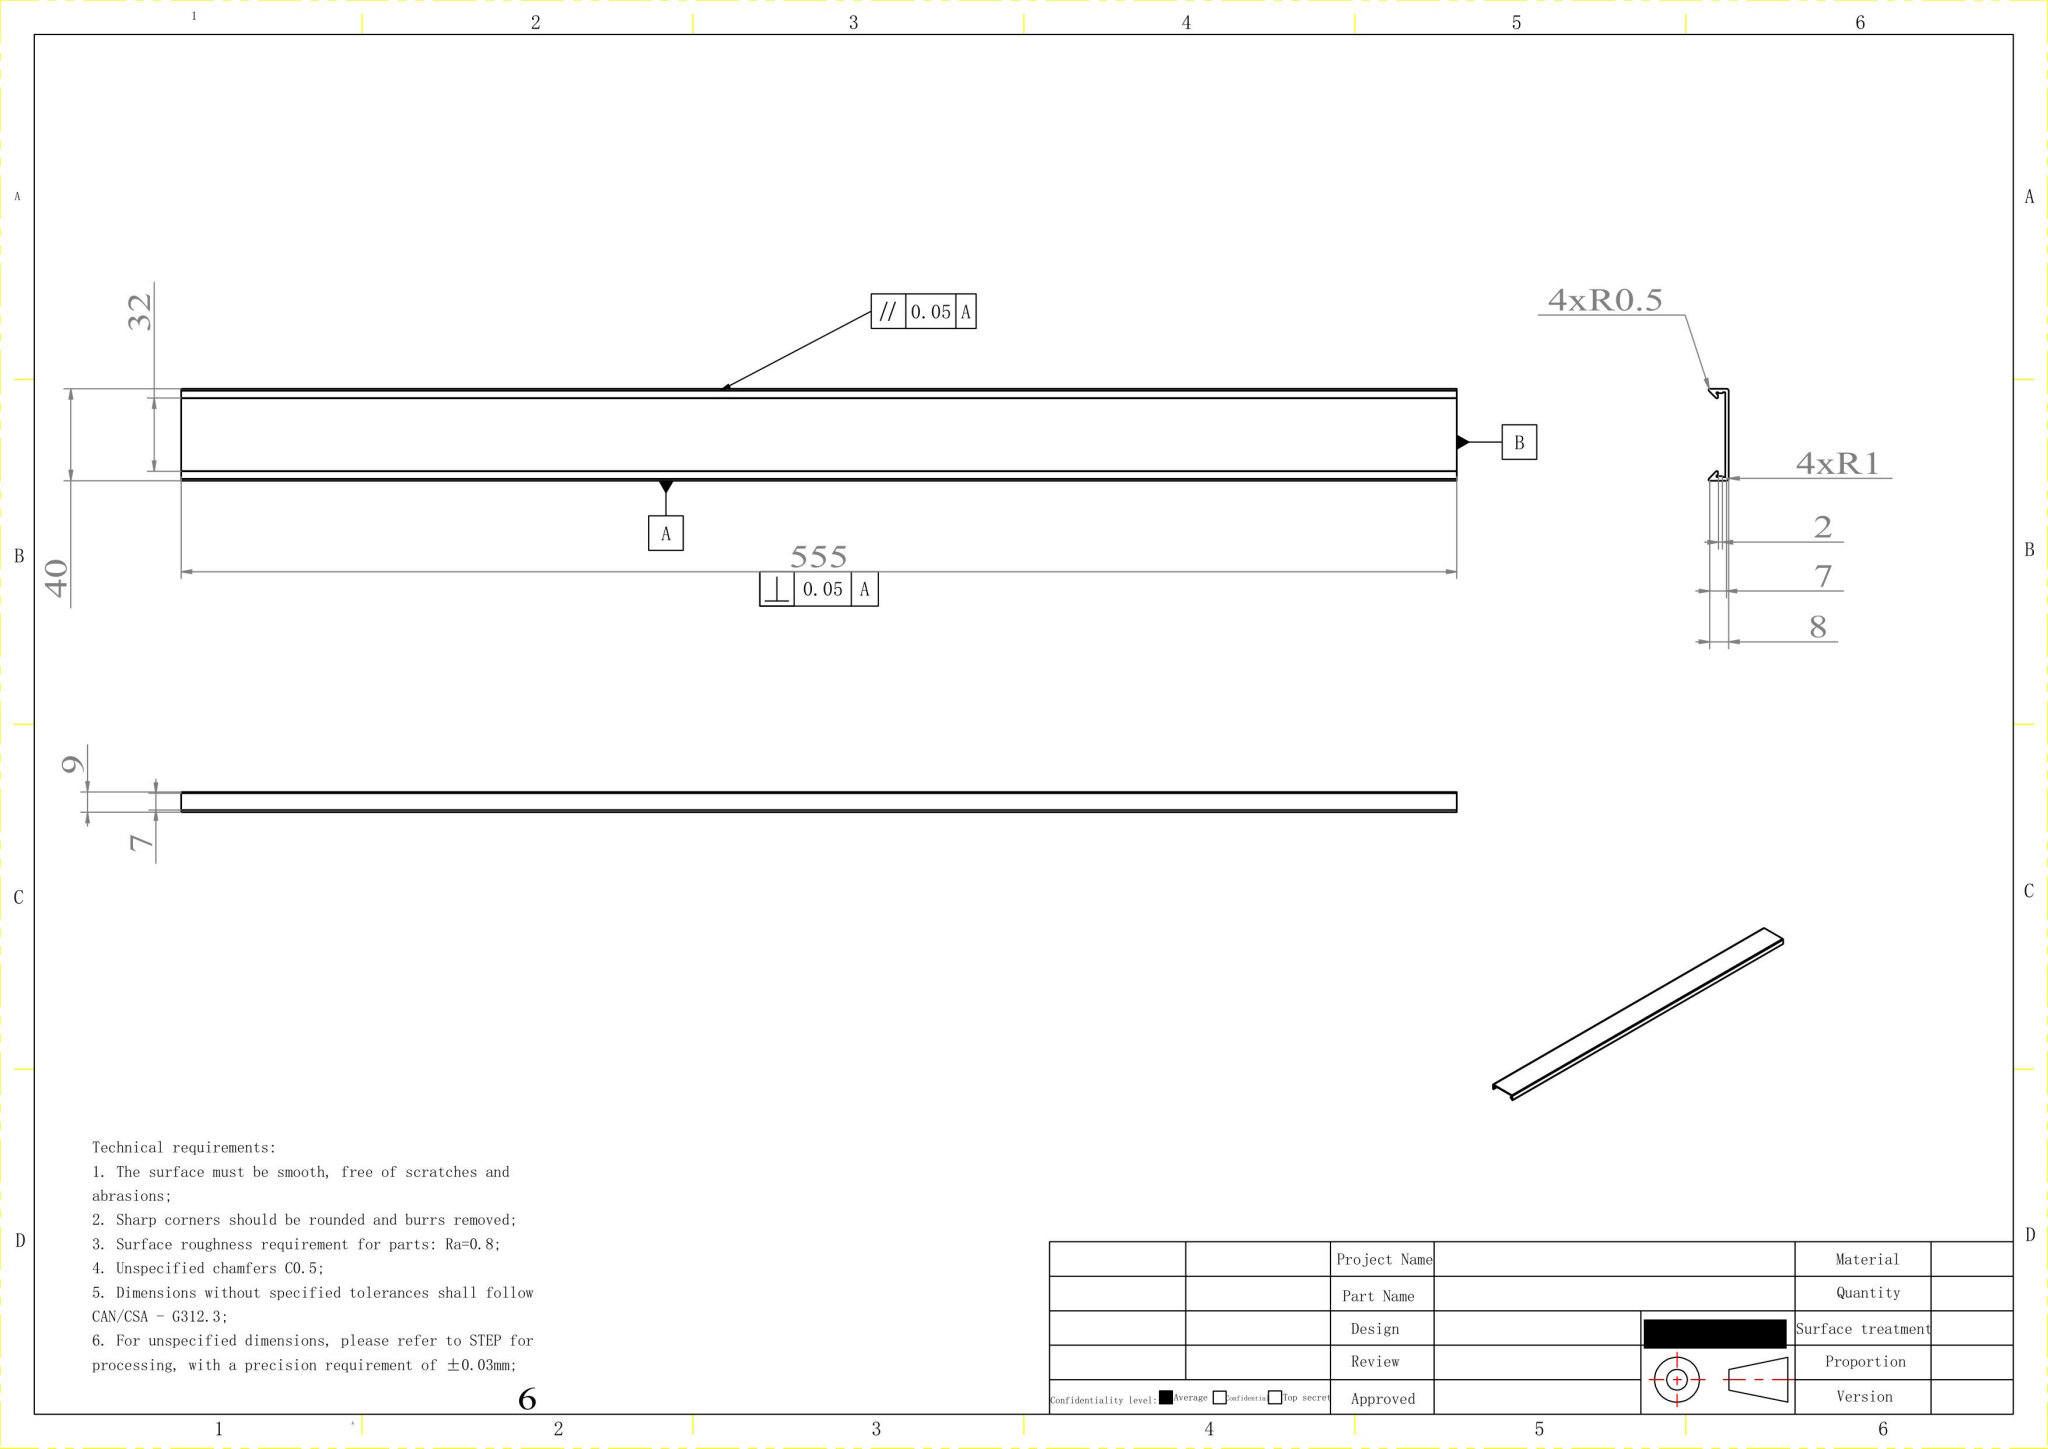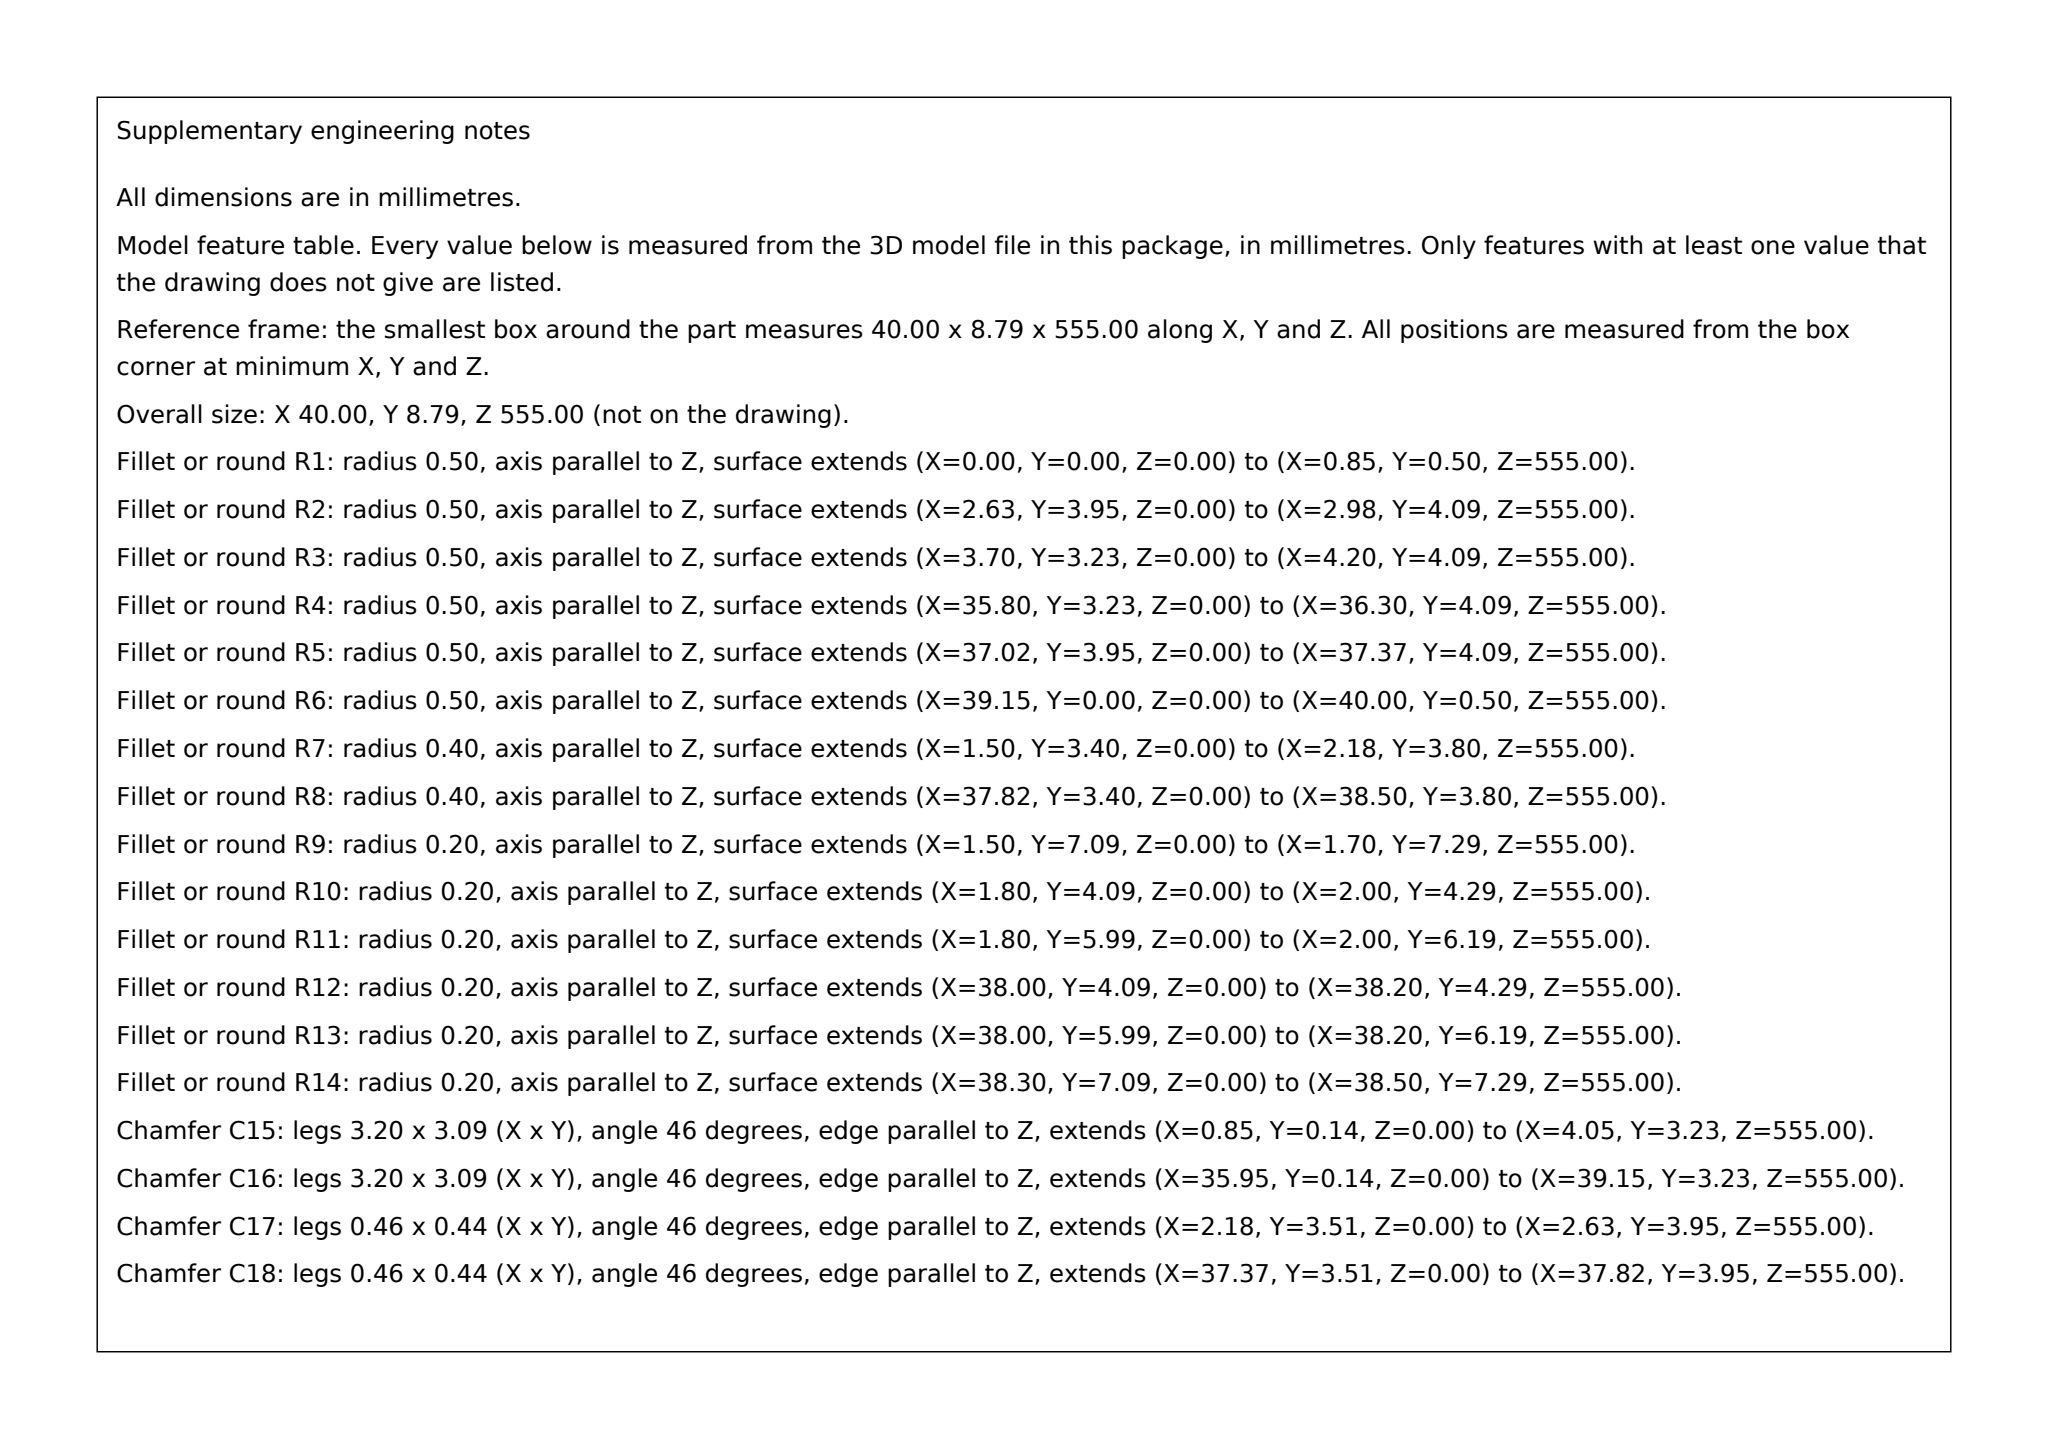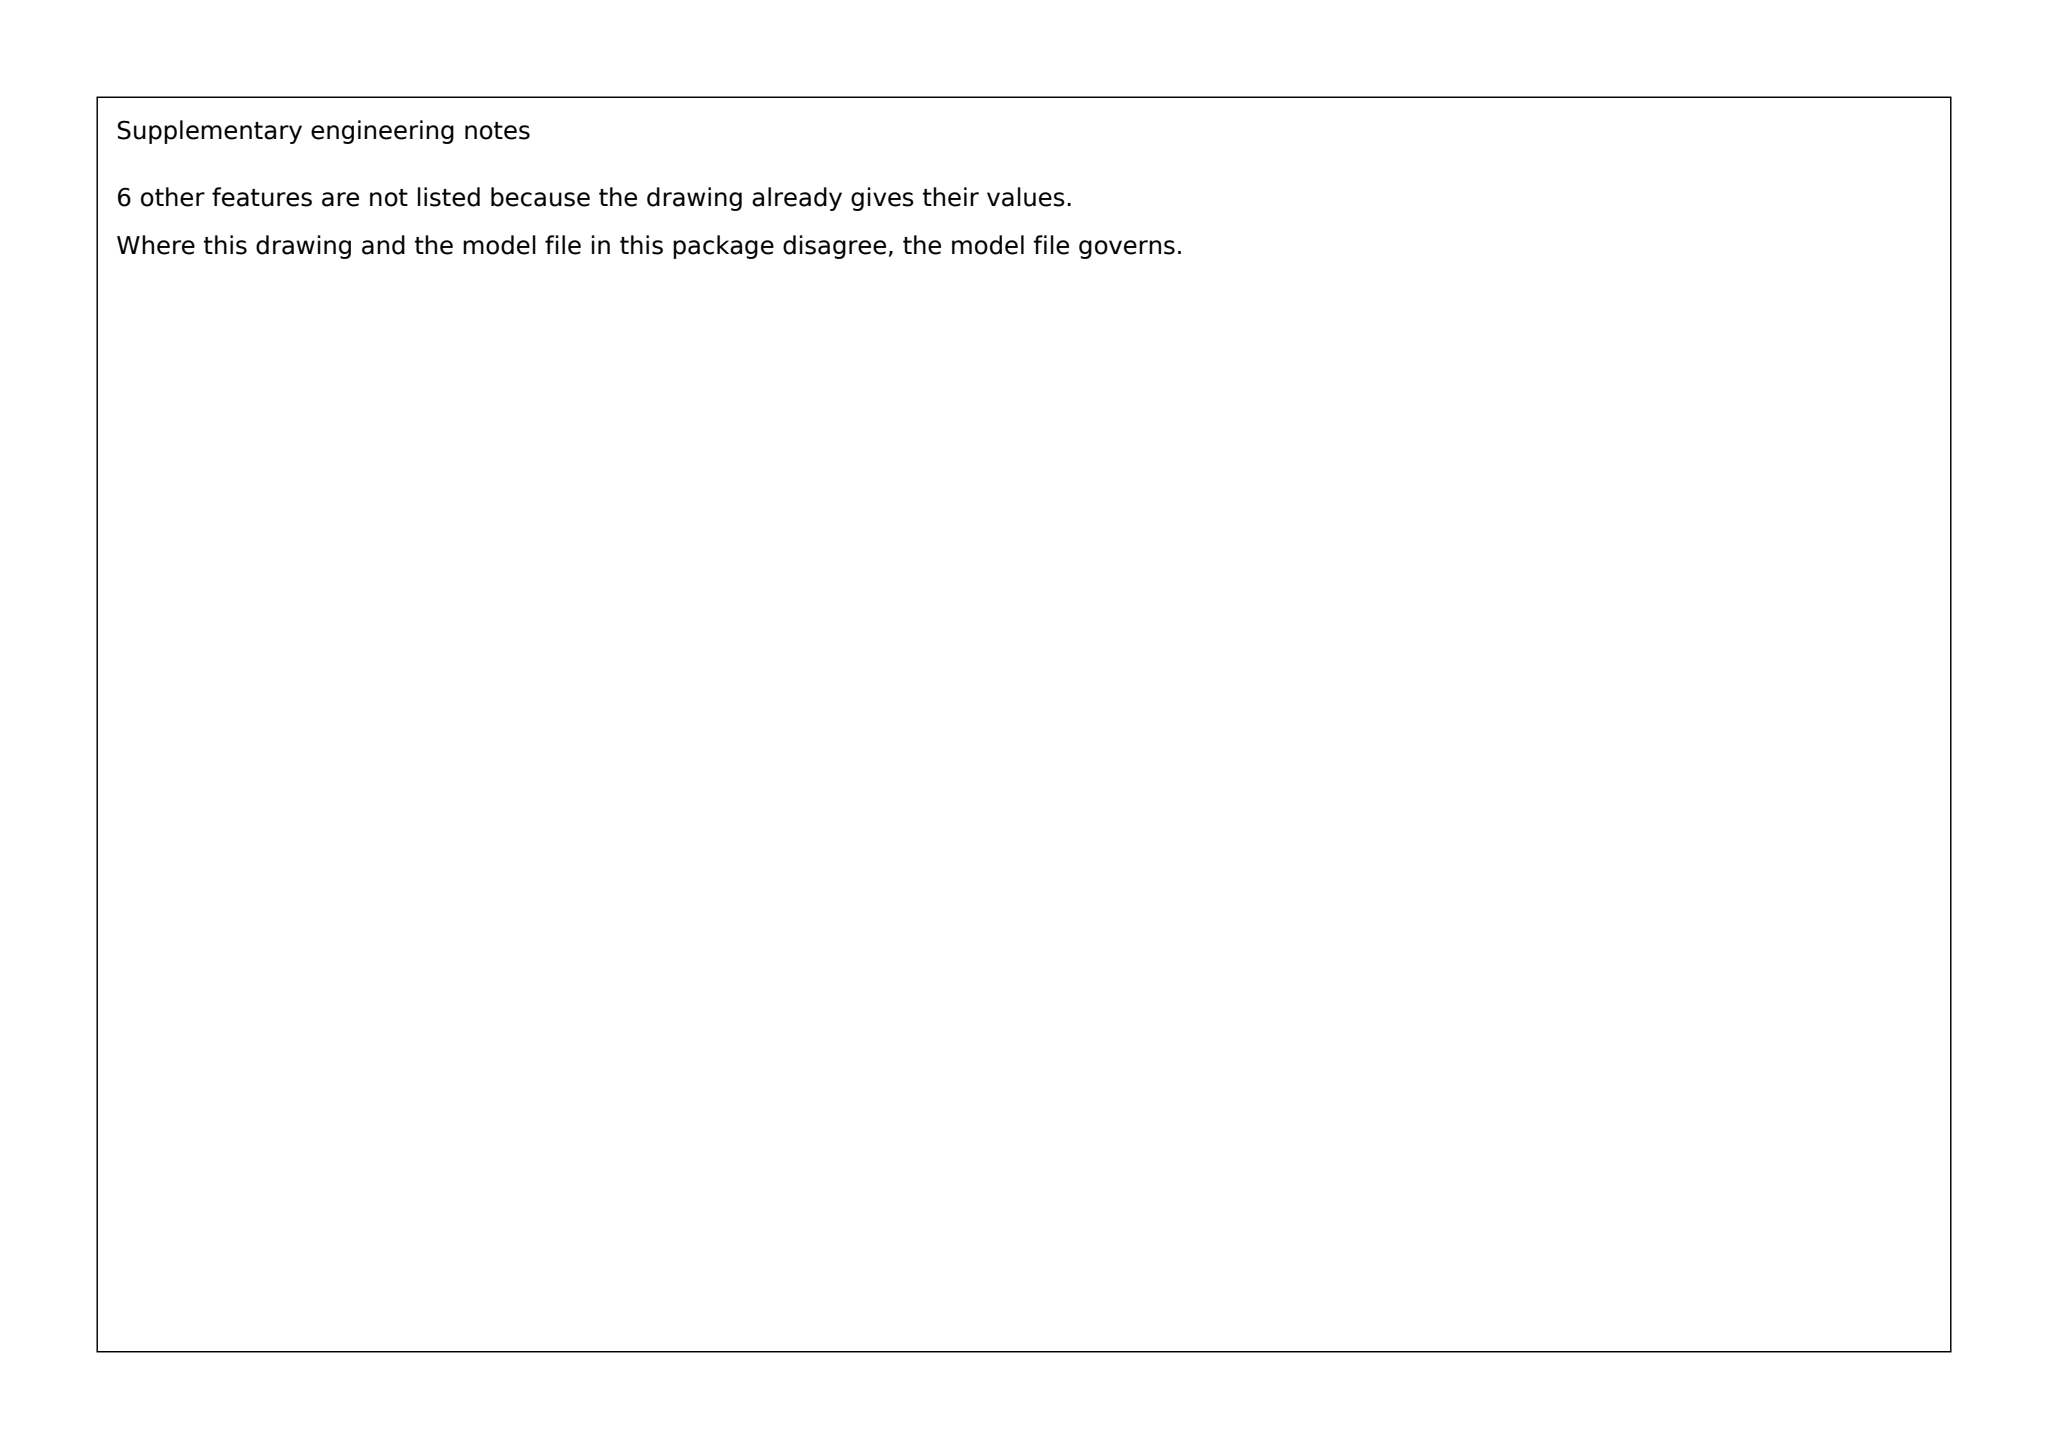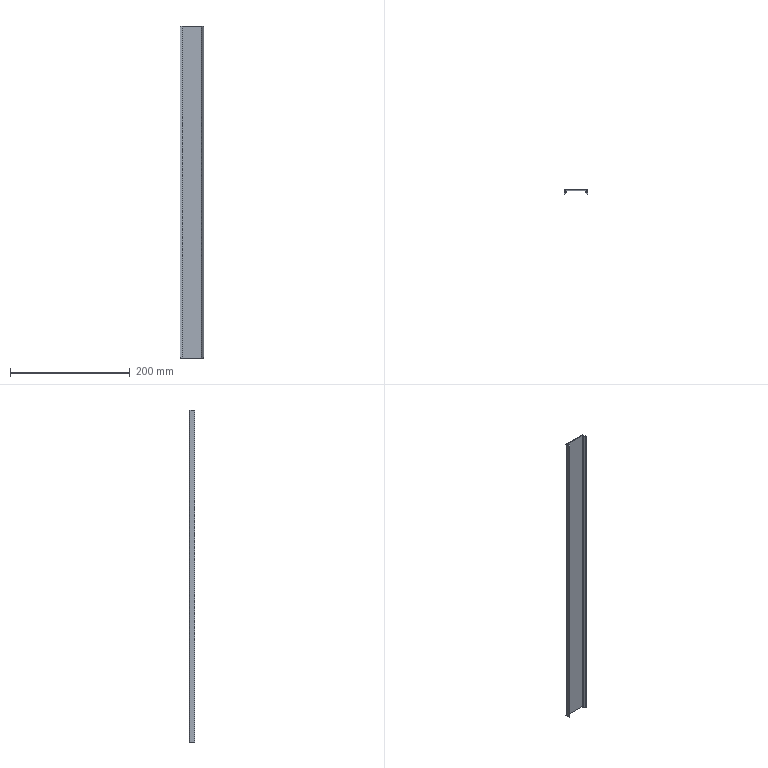Part | SolidWorks | mm | 1 solid | 42 faces | box 40 x 8.79 x 555 mm | volume 51260 mm3 | plane 22 | cylinder 20 | commonest cylinder face diameters 0.4 x6 1 x6 0.2 x4 0.8 x2 2 x2